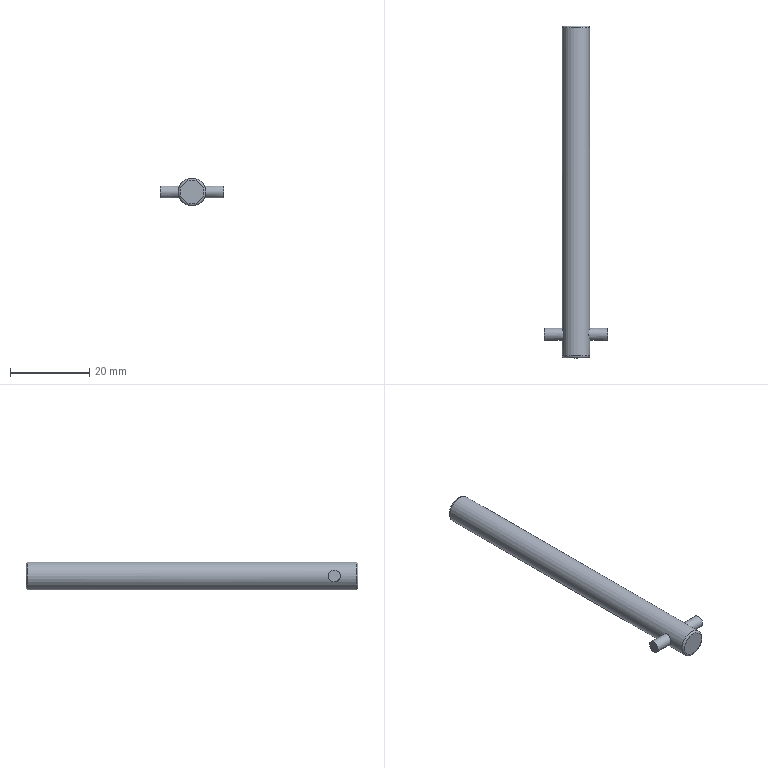Component | NX | FLYWHEEL_SHAFT | 1 solid | 9 faces | volume 3295 mm3 | plane 4 | cylinder 3 | torus 2 | commonest cylinder face diameters 3 x2 7 x1